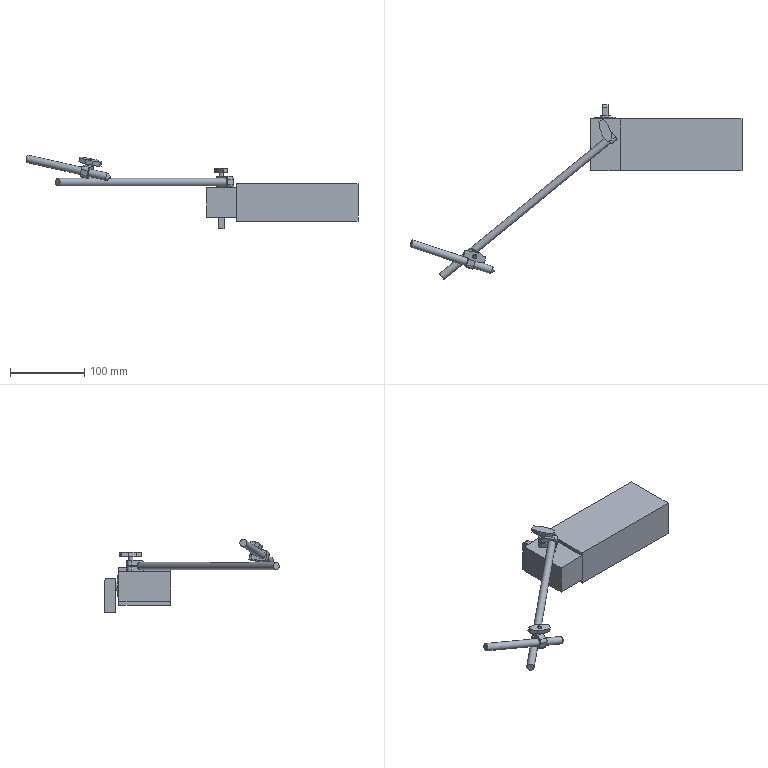Assembly | NX | mm | 8 component files | 11 solids | 95 faces | box 447.34 x 235.09 x 99.2 mm | volume 733461 mm3 | plane 67 | cylinder 27 | cone 1 | commonest cylinder face diameters 8 x13 6 x7 10 x5 28.3 x1 13.052 x1
Bill of materials:
unnamed part 1 | 1 |  | Rectangular box-shaped body with a small round hole on its top face. A short stepped cylindrical shaft sticks out from one end face, and a thin rectangular plate with one rounded corner sits at the end of the shaft.
unnamed part 2 | 1 |  | Long, thin, straight solid cylindrical rod with flat ends.
unnamed part 3 | 1 |  | Plain solid rectangular block with no visible holes, cutouts or edge rounding.
unnamed part 4 | 1 |  | Flat plate with an elongated six-sided outline: two parallel long sides and tapered ends. A single round through-hole is in the middle, and a short cylindrical boss on the underside lines up with the hole.
unnamed part 5 | 1 |  | Straight cylindrical pin with a chamfered, cone-shaped tip at one end and a flat or slightly rounded opposite end.
unnamed part 6 | 2 |  | Split clamp block with rounded ends. A large round bore runs through one end, and a slot runs from the bore to the opposite end, dividing that end into two jaws. A smaller cross-hole passes through both jaws, roughly perpendicular to the slot.
unnamed part 7 | 1 |  | T-shaped part: a flat head plate with an elongated six-sided (stretched hexagon) outline, with a straight cylindrical stem coming out of the center of one face.
Mates:
1. concentric | Manual_Nut 1 arc | Block_1 1 arc
2. bond | Gauge_Rod_1 1 component | Block_1 2 component
3. bond | Manual_Screw 1 component | Block_1 2 component
4. fix | Block_1 2 component
5. fix | Manual_Screw 1 component
6. fix | Gauge_Rod_1 1 component
7. distance | Mag_Base 1 face | Pen_Holder_Block 1 face
8. center | Mag_Base 1 face | Mag_Base 1 face | Pen_Holder_Block 1 face | Pen_Holder_Block 1 face
9. distance | Mag_Base 1 face | Pen_Holder_Block 1 face